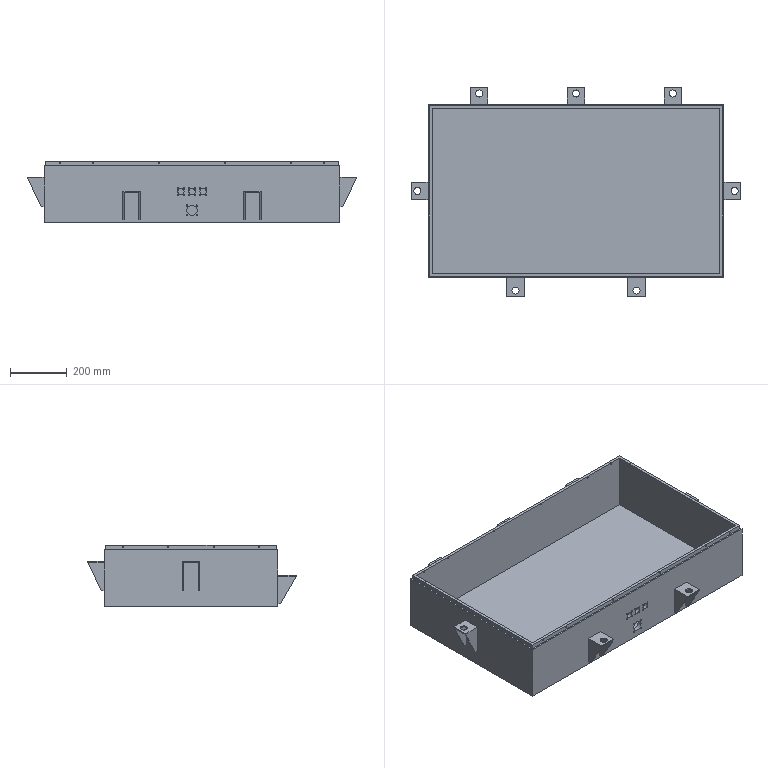Component | NX | ENCLOSURE | 1 solid | 140 faces | volume 19230413 mm3 | plane 93 | cylinder 47 | commonest cylinder face diameters 4 x36 25 x7 22.2 x3 36.5 x1